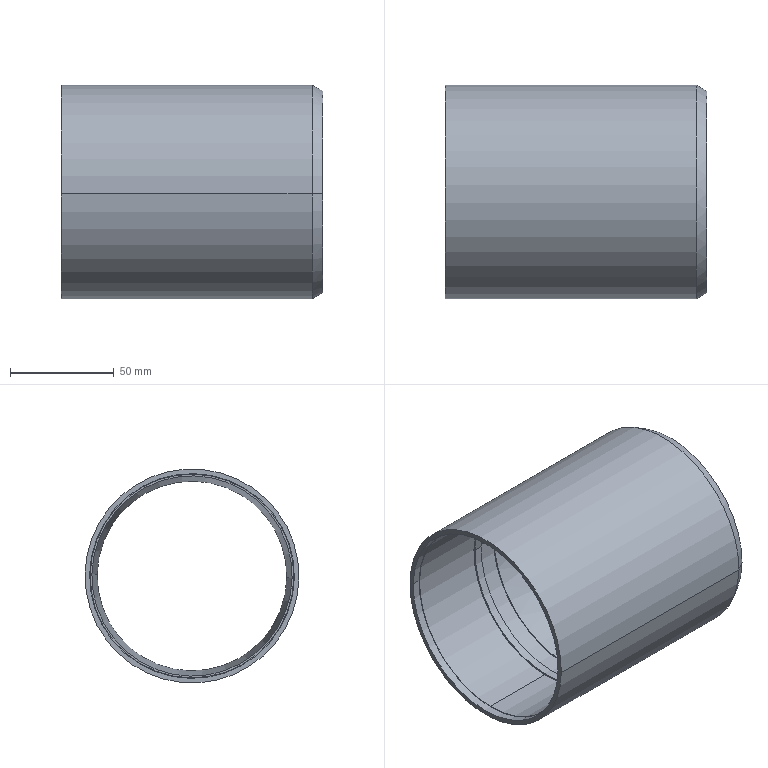Component | SolidWorks | 216InnerTubeAssembly-1_SnapRingSeat-1 | 1 solid | 24 faces | box 126 x 103 x 103 mm | volume 139518 mm3 | cylinder 10 | cone 8 | plane 6 | commonest cylinder face diameters 98.01 x2 98.4 x2 98.539 x2 103 x2 96.4 x2 | material Alloy Steel
build123d program:
from build123d import *

# Parameters (mm, degrees)
SKETCH1_W = 37.278
SKETCH1_H = 1.505


with BuildPart() as part:
    # Model → Revolve1 (revolve)
    with BuildSketch(Plane.XY, mode=Mode.PRIVATE) as revolve1_sk:
        Polygon((-1.168, 45.275), (-0.1676, 46.275), (-0.1676, 48.084), (-5.364, 51.084), (-126.168, 51.084), (-126.168, 48.853), (-122.168, 48.853), (-122.168, 47.784), (-81.168, 47.784), (-81.168, 48.784), (-71.668, 48.784), (-71.668, 48.284), (-8.168, 45.243), align=None)
    revolve(revolve1_sk.sketch.rotate(Axis((-130.696, -0.4163, 0), (1, 0, 0)), 180), axis=Axis((-130.696, -0.4163, 0), (1, 0, 0)))

    # Sketch1 → Cut-Revolve1 (revolve, cut)
    with BuildSketch(Plane.XY, mode=Mode.PRIVATE) as cut_revolve1_sk:
        with Locations((-103.806, 47.836)):
            Rectangle(SKETCH1_W, SKETCH1_H)
    revolve(cut_revolve1_sk.sketch.rotate(Axis((-127.445, -0.4163, 0), (1, 0, 0)), 180), axis=Axis((-127.445, -0.4163, 0), (1, 0, 0)), mode=Mode.SUBTRACT)


solid = part.part

# Placed as in the assembly
solid = solid.moved(Location((2974.445, 0.4163, 0), (0, 0, 0)))
STEP:
#1=CARTESIAN_POINT('',(113.751,0.03464,-1.929));
#2=VERTEX_POINT('',#1);
#3=CARTESIAN_POINT('',(113.751,-0.03464,1.929));
#4=VERTEX_POINT('',#3);
#5=CARTESIAN_POINT('',(113.751,-0.,0.));
#6=DIRECTION('',(-1.,-0.,0.));
#7=DIRECTION('',(0.,-0.01796,0.9998));
#8=AXIS2_PLACEMENT_3D('',#5,#6,#7);
#9=CIRCLE('',#8,1.929);
#10=EDGE_CURVE('',#2,#4,#9,.T.);
#11=ORIENTED_EDGE('',*,*,#10,.F.);
#12=CARTESIAN_POINT('',(112.294,0.03464,-1.929));
#13=VERTEX_POINT('',#12);
#14=CARTESIAN_POINT('',(112.087,0.03464,-1.929));
#15=DIRECTION('',(-1.,-0.,0.));
#16=VECTOR('',#15,39.37);
#17=LINE('',#14,#16);
#18=EDGE_CURVE('',#2,#13,#17,.T.);
#19=ORIENTED_EDGE('',*,*,#18,.T.);
#20=CARTESIAN_POINT('',(112.294,-0.03464,1.929));
#21=VERTEX_POINT('',#20);
#22=CARTESIAN_POINT('',(112.294,-0.,0.));
#23=DIRECTION('',(1.,0.,0.));
#24=DIRECTION('',(0.,-0.9998,-0.01796));
#25=AXIS2_PLACEMENT_3D('',#22,#23,#24);
#26=CIRCLE('',#25,1.929);
#27=EDGE_CURVE('',#21,#13,#26,.T.);
#28=ORIENTED_EDGE('',*,*,#27,.F.);
#29=CARTESIAN_POINT('',(112.087,-0.03464,1.929));
#30=DIRECTION('',(-1.,-0.,0.));
#31=VECTOR('',#30,39.37);
#32=LINE('',#29,#31);
#33=EDGE_CURVE('',#4,#21,#32,.T.);
#34=ORIENTED_EDGE('',*,*,#33,.F.);
#35=EDGE_LOOP('',(#11,#19,#28,#34));
#36=FACE_OUTER_BOUND('',#35,.T.);
#37=CARTESIAN_POINT('',(112.087,-0.,0.));
#38=DIRECTION('',(-1.,-0.,0.));
#39=DIRECTION('',(0.,-0.01796,0.9998));
#40=AXIS2_PLACEMENT_3D('',#37,#38,#39);
#41=CYLINDRICAL_SURFACE('',#40,1.929);
#42=ADVANCED_FACE('',(#36),#41,.F.);
#43=CARTESIAN_POINT('',(116.783,1.797,0.03228));
#44=VERTEX_POINT('',#43);
#45=CARTESIAN_POINT('',(116.783,-1.797,-0.03228));
#46=VERTEX_POINT('',#45);
#47=CARTESIAN_POINT('',(116.783,-0.,0.));
#48=DIRECTION('',(-1.,-0.,-0.));
#49=DIRECTION('',(0.,-0.9998,-0.01796));
#50=AXIS2_PLACEMENT_3D('',#47,#48,#49);
#51=CIRCLE('',#50,1.798);
#52=EDGE_CURVE('',#44,#46,#51,.T.);
#53=ORIENTED_EDGE('',*,*,#52,.T.);
#54=CARTESIAN_POINT('',(117.058,-1.799,-0.0323));
#55=VERTEX_POINT('',#54);
#56=CARTESIAN_POINT('',(116.783,-1.797,-0.03228));
#57=DIRECTION('',(1.,-0.004511,-0.00008102));
#58=VECTOR('',#57,39.37);
#59=LINE('',#56,#58);
#60=EDGE_CURVE('',#46,#55,#59,.T.);
#61=ORIENTED_EDGE('',*,*,#60,.T.);
#62=CARTESIAN_POINT('',(117.058,1.799,0.0323));
#63=VERTEX_POINT('',#62);
#64=CARTESIAN_POINT('',(117.058,-0.,0.));
#65=DIRECTION('',(-1.,-0.,-0.));
#66=DIRECTION('',(0.,-0.9998,-0.01796));
#67=AXIS2_PLACEMENT_3D('',#64,#65,#66);
#68=CIRCLE('',#67,1.799);
#69=EDGE_CURVE('',#63,#55,#68,.T.);
#70=ORIENTED_EDGE('',*,*,#69,.F.);
#71=CARTESIAN_POINT('',(116.783,1.797,0.03228));
#72=DIRECTION('',(1.,0.004511,0.00008102));
#73=VECTOR('',#72,39.37);
#74=LINE('',#71,#73);
#75=EDGE_CURVE('',#44,#63,#74,.T.);
#76=ORIENTED_EDGE('',*,*,#75,.F.);
#77=EDGE_LOOP('',(#53,#61,#70,#76));
#78=FACE_OUTER_BOUND('',#77,.T.);
#79=CARTESIAN_POINT('',(116.783,-0.,0.));
#80=DIRECTION('',(1.,0.,0.));
#81=DIRECTION('',(0.,0.9998,0.01796));
#82=AXIS2_PLACEMENT_3D('',#79,#80,#81);
#83=CONICAL_SURFACE('',#82,1.798,0.004512);
#84=ADVANCED_FACE('',(#78),#83,.F.);
#85=ORIENTED_EDGE('',*,*,#52,.F.);
#86=CARTESIAN_POINT('',(114.283,1.917,0.03443));
#87=VERTEX_POINT('',#86);
#88=CARTESIAN_POINT('',(116.783,1.797,0.03228));
#89=DIRECTION('',(-0.9989,0.04782,0.0008588));
#90=VECTOR('',#89,39.37);
#91=LINE('',#88,#90);
#92=EDGE_CURVE('',#44,#87,#91,.T.);
#93=ORIENTED_EDGE('',*,*,#92,.T.);
#94=CARTESIAN_POINT('',(114.283,-1.917,-0.03443));
#95=VERTEX_POINT('',#94);
#96=CARTESIAN_POINT('',(114.283,-0.,0.));
#97=DIRECTION('',(-1.,-0.,-0.));
#98=DIRECTION('',(0.,-0.9998,-0.01796));
#99=AXIS2_PLACEMENT_3D('',#96,#97,#98);
#100=CIRCLE('',#99,1.917);
#101=EDGE_CURVE('',#87,#95,#100,.T.);
#102=ORIENTED_EDGE('',*,*,#101,.T.);
#103=CARTESIAN_POINT('',(116.783,-1.797,-0.03228));
#104=DIRECTION('',(-0.9989,-0.04782,-0.0008588));
#105=VECTOR('',#104,39.37);
#106=LINE('',#103,#105);
#107=EDGE_CURVE('',#46,#95,#106,.T.);
#108=ORIENTED_EDGE('',*,*,#107,.F.);
#109=EDGE_LOOP('',(#85,#93,#102,#108));
#110=FACE_OUTER_BOUND('',#109,.T.);
#111=CARTESIAN_POINT('',(116.783,-0.,0.));
#112=DIRECTION('',(-1.,-0.,-0.));
#113=DIRECTION('',(0.,-0.9998,-0.01796));
#114=AXIS2_PLACEMENT_3D('',#111,#112,#113);
#115=CONICAL_SURFACE('',#114,1.798,0.04785);
#116=ADVANCED_FACE('',(#110),#115,.F.);
#117=CARTESIAN_POINT('',(114.283,1.937,0.03478));
#118=VERTEX_POINT('',#117);
#119=CARTESIAN_POINT('',(114.283,-1.937,-0.03478));
#120=VERTEX_POINT('',#119);
#121=CARTESIAN_POINT('',(114.283,-0.,0.));
#122=DIRECTION('',(-1.,-0.,-0.));
#123=DIRECTION('',(0.,-0.9998,-0.01796));
#124=AXIS2_PLACEMENT_3D('',#121,#122,#123);
#125=CIRCLE('',#124,1.937);
#126=EDGE_CURVE('',#118,#120,#125,.T.);
#127=ORIENTED_EDGE('',*,*,#126,.F.);
#128=CARTESIAN_POINT('',(113.909,1.937,0.03478));
#129=VERTEX_POINT('',#128);
#130=CARTESIAN_POINT('',(111.959,1.937,0.03478));
#131=DIRECTION('',(-1.,-0.,-0.));
#132=VECTOR('',#131,39.37);
#133=LINE('',#130,#132);
#134=EDGE_CURVE('',#118,#129,#133,.T.);
#135=ORIENTED_EDGE('',*,*,#134,.T.);
#136=CARTESIAN_POINT('',(113.909,-1.937,-0.03478));
#137=VERTEX_POINT('',#136);
#138=CARTESIAN_POINT('',(113.909,-0.,0.));
#139=DIRECTION('',(-1.,-0.,-0.));
#140=DIRECTION('',(0.,-0.9998,-0.01796));
#141=AXIS2_PLACEMENT_3D('',#138,#139,#140);
#142=CIRCLE('',#141,1.937);
#143=EDGE_CURVE('',#129,#137,#142,.T.);
#144=ORIENTED_EDGE('',*,*,#143,.T.);
#145=CARTESIAN_POINT('',(111.959,-1.937,-0.03478));
#146=DIRECTION('',(-1.,-0.,-0.));
#147=VECTOR('',#146,39.37);
#148=LINE('',#145,#147);
#149=EDGE_CURVE('',#120,#137,#148,.T.);
#150=ORIENTED_EDGE('',*,*,#149,.F.);
#151=EDGE_LOOP('',(#127,#135,#144,#150));
#152=FACE_OUTER_BOUND('',#151,.T.);
#153=CARTESIAN_POINT('',(111.959,-0.,0.));
#154=DIRECTION('',(-1.,-0.,-0.));
#155=DIRECTION('',(0.,-0.9998,-0.01796));
#156=AXIS2_PLACEMENT_3D('',#153,#154,#155);
#157=CYLINDRICAL_SURFACE('',#156,1.937);
#158=ADVANCED_FACE('',(#152),#157,.F.);
#159=CARTESIAN_POINT('',(112.294,1.939,0.03483));
#160=VERTEX_POINT('',#159);
#161=CARTESIAN_POINT('',(112.294,-1.939,-0.03483));
#162=VERTEX_POINT('',#161);
#163=CARTESIAN_POINT('',(112.294,-0.,0.));
#164=DIRECTION('',(-1.,-0.,-0.));
#165=DIRECTION('',(0.,-0.9998,-0.01796));
#166=AXIS2_PLACEMENT_3D('',#163,#164,#165);
#167=CIRCLE('',#166,1.94);
#168=EDGE_CURVE('',#160,#162,#167,.T.);
#169=ORIENTED_EDGE('',*,*,#168,.F.);
#170=CARTESIAN_POINT('',(112.137,1.939,0.03483));
#171=VERTEX_POINT('',#170);
#172=CARTESIAN_POINT('',(111.959,1.939,0.03483));
#173=DIRECTION('',(-1.,-0.,-0.));
#174=VECTOR('',#173,39.37);
#175=LINE('',#172,#174);
#176=EDGE_CURVE('',#160,#171,#175,.T.);
#177=ORIENTED_EDGE('',*,*,#176,.T.);
#178=CARTESIAN_POINT('',(112.137,-1.939,-0.03483));
#179=VERTEX_POINT('',#178);
#180=CARTESIAN_POINT('',(112.137,-0.,0.));
#181=DIRECTION('',(-1.,-0.,-0.));
#182=DIRECTION('',(0.,-0.9998,-0.01796));
#183=AXIS2_PLACEMENT_3D('',#180,#181,#182);
#184=CIRCLE('',#183,1.94);
#185=EDGE_CURVE('',#171,#179,#184,.T.);
#186=ORIENTED_EDGE('',*,*,#185,.T.);
#187=CARTESIAN_POINT('',(111.959,-1.939,-0.03483));
#188=DIRECTION('',(-1.,-0.,-0.));
#189=VECTOR('',#188,39.37);
#190=LINE('',#187,#189);
#191=EDGE_CURVE('',#162,#179,#190,.T.);
#192=ORIENTED_EDGE('',*,*,#191,.F.);
#193=EDGE_LOOP('',(#169,#177,#186,#192));
#194=FACE_OUTER_BOUND('',#193,.T.);
#195=CARTESIAN_POINT('',(111.959,-0.,0.));
#196=DIRECTION('',(-1.,-0.,-0.));
#197=DIRECTION('',(0.,-0.9998,-0.01796));
#198=AXIS2_PLACEMENT_3D('',#195,#196,#197);
#199=CYLINDRICAL_SURFACE('',#198,1.94);
#200=ADVANCED_FACE('',(#194),#199,.F.);
#201=CARTESIAN_POINT('',(116.893,-2.027,-0.03641));
#202=VERTEX_POINT('',#201);
#203=CARTESIAN_POINT('',(116.893,2.027,0.03641));
#204=VERTEX_POINT('',#203);
#205=CARTESIAN_POINT('',(116.893,-0.,0.));
#206=DIRECTION('',(-1.,-0.,-0.));
#207=DIRECTION('',(0.,-0.9998,-0.01796));
#208=AXIS2_PLACEMENT_3D('',#205,#206,#207);
#209=CIRCLE('',#208,2.028);
#210=EDGE_CURVE('',#202,#204,#209,.T.);
#211=ORIENTED_EDGE('',*,*,#210,.T.);
#212=CARTESIAN_POINT('',(112.137,2.027,0.03641));
#213=VERTEX_POINT('',#212);
#214=CARTESIAN_POINT('',(111.959,2.027,0.03641));
#215=DIRECTION('',(-1.,-0.,-0.));
#216=VECTOR('',#215,39.37);
#217=LINE('',#214,#216);
#218=EDGE_CURVE('',#204,#213,#217,.T.);
#219=ORIENTED_EDGE('',*,*,#218,.T.);
#220=CARTESIAN_POINT('',(112.137,-2.027,-0.03641));
#221=VERTEX_POINT('',#220);
#222=CARTESIAN_POINT('',(112.137,-0.,0.));
#223=DIRECTION('',(-1.,-0.,-0.));
#224=DIRECTION('',(0.,-0.9998,-0.01796));
#225=AXIS2_PLACEMENT_3D('',#222,#223,#224);
#226=CIRCLE('',#225,2.028);
#227=EDGE_CURVE('',#221,#213,#226,.T.);
#228=ORIENTED_EDGE('',*,*,#227,.F.);
#229=CARTESIAN_POINT('',(111.959,-2.027,-0.03641));
#230=DIRECTION('',(-1.,-0.,-0.));
#231=VECTOR('',#230,39.37);
#232=LINE('',#229,#231);
#233=EDGE_CURVE('',#202,#221,#232,.T.);
#234=ORIENTED_EDGE('',*,*,#233,.F.);
#235=EDGE_LOOP('',(#211,#219,#228,#234));
#236=FACE_OUTER_BOUND('',#235,.T.);
#237=CARTESIAN_POINT('',(111.959,-0.,0.));
#238=DIRECTION('',(-1.,-0.,-0.));
#239=DIRECTION('',(0.,-0.9998,-0.01796));
#240=AXIS2_PLACEMENT_3D('',#237,#238,#239);
#241=CYLINDRICAL_SURFACE('',#240,2.028);
#242=ADVANCED_FACE('',(#236),#241,.T.);
#243=CARTESIAN_POINT('',(117.098,-1.909,-0.03429));
#244=VERTEX_POINT('',#243);
#245=CARTESIAN_POINT('',(117.098,1.909,0.03429));
#246=VERTEX_POINT('',#245);
#247=CARTESIAN_POINT('',(117.098,-0.,0.));
#248=DIRECTION('',(-1.,-0.,-0.));
#249=DIRECTION('',(0.,-0.9998,-0.01796));
#250=AXIS2_PLACEMENT_3D('',#247,#248,#249);
#251=CIRCLE('',#250,1.909);
#252=EDGE_CURVE('',#244,#246,#251,.T.);
#253=ORIENTED_EDGE('',*,*,#252,.T.);
#254=CARTESIAN_POINT('',(117.098,1.909,0.03429));
#255=DIRECTION('',(-0.866,0.4999,0.008978));
#256=VECTOR('',#255,39.37);
#257=LINE('',#254,#256);
#258=EDGE_CURVE('',#246,#204,#257,.T.);
#259=ORIENTED_EDGE('',*,*,#258,.T.);
#260=ORIENTED_EDGE('',*,*,#210,.F.);
#261=CARTESIAN_POINT('',(117.098,-1.909,-0.03429));
#262=DIRECTION('',(-0.866,-0.4999,-0.008978));
#263=VECTOR('',#262,39.37);
#264=LINE('',#261,#263);
#265=EDGE_CURVE('',#244,#202,#264,.T.);
#266=ORIENTED_EDGE('',*,*,#265,.F.);
#267=EDGE_LOOP('',(#253,#259,#260,#266));
#268=FACE_OUTER_BOUND('',#267,.T.);
#269=CARTESIAN_POINT('',(117.098,-0.,0.));
#270=DIRECTION('',(-1.,-0.,-0.));
#271=DIRECTION('',(0.,-0.9998,-0.01796));
#272=AXIS2_PLACEMENT_3D('',#269,#270,#271);
#273=CONICAL_SURFACE('',#272,1.909,0.5236);
#274=ADVANCED_FACE('',(#268),#273,.T.);
#275=ORIENTED_EDGE('',*,*,#69,.T.);
#276=CARTESIAN_POINT('',(117.098,-1.838,-0.03301));
#277=VERTEX_POINT('',#276);
#278=CARTESIAN_POINT('',(117.058,-1.799,-0.0323));
#279=DIRECTION('',(0.7071,-0.707,-0.0127));
#280=VECTOR('',#279,39.37);
#281=LINE('',#278,#280);
#282=EDGE_CURVE('',#55,#277,#281,.T.);
#283=ORIENTED_EDGE('',*,*,#282,.T.);
#284=CARTESIAN_POINT('',(117.098,1.838,0.03301));
#285=VERTEX_POINT('',#284);
#286=CARTESIAN_POINT('',(117.098,-0.,0.));
#287=DIRECTION('',(-1.,-0.,-0.));
#288=DIRECTION('',(0.,-0.9998,-0.01796));
#289=AXIS2_PLACEMENT_3D('',#286,#287,#288);
#290=CIRCLE('',#289,1.838);
#291=EDGE_CURVE('',#285,#277,#290,.T.);
#292=ORIENTED_EDGE('',*,*,#291,.F.);
#293=CARTESIAN_POINT('',(117.058,1.799,0.0323));
#294=DIRECTION('',(0.7071,0.707,0.0127));
#295=VECTOR('',#294,39.37);
#296=LINE('',#293,#295);
#297=EDGE_CURVE('',#63,#285,#296,.T.);
#298=ORIENTED_EDGE('',*,*,#297,.F.);
#299=EDGE_LOOP('',(#275,#283,#292,#298));
#300=FACE_OUTER_BOUND('',#299,.T.);
#301=CARTESIAN_POINT('',(117.058,-0.,0.));
#302=DIRECTION('',(1.,0.,0.));
#303=DIRECTION('',(0.,0.9998,0.01796));
#304=AXIS2_PLACEMENT_3D('',#301,#302,#303);
#305=CONICAL_SURFACE('',#304,1.799,0.7854);
#306=ADVANCED_FACE('',(#300),#305,.F.);
#307=CARTESIAN_POINT('',(113.909,1.897,0.03407));
#308=VERTEX_POINT('',#307);
#309=CARTESIAN_POINT('',(113.909,-1.897,-0.03407));
#310=VERTEX_POINT('',#309);
#311=CARTESIAN_POINT('',(113.909,-0.,0.));
#312=DIRECTION('',(-1.,-0.,-0.));
#313=DIRECTION('',(0.,-0.9998,-0.01796));
#314=AXIS2_PLACEMENT_3D('',#311,#312,#313);
#315=CIRCLE('',#314,1.898);
#316=EDGE_CURVE('',#308,#310,#315,.T.);
#317=ORIENTED_EDGE('',*,*,#316,.F.);
#318=CARTESIAN_POINT('',(113.751,1.897,0.03407));
#319=VERTEX_POINT('',#318);
#320=CARTESIAN_POINT('',(111.959,1.897,0.03407));
#321=DIRECTION('',(-1.,-0.,-0.));
#322=VECTOR('',#321,39.37);
#323=LINE('',#320,#322);
#324=EDGE_CURVE('',#308,#319,#323,.T.);
#325=ORIENTED_EDGE('',*,*,#324,.T.);
#326=CARTESIAN_POINT('',(113.751,-1.897,-0.03407));
#327=VERTEX_POINT('',#326);
#328=CARTESIAN_POINT('',(113.751,-0.,0.));
#329=DIRECTION('',(-1.,-0.,0.));
#330=DIRECTION('',(0.,-0.01796,0.9998));
#331=AXIS2_PLACEMENT_3D('',#328,#329,#330);
#332=CIRCLE('',#331,1.898);
#333=EDGE_CURVE('',#319,#327,#332,.T.);
#334=ORIENTED_EDGE('',*,*,#333,.T.);
#335=CARTESIAN_POINT('',(111.959,-1.897,-0.03407));
#336=DIRECTION('',(-1.,-0.,-0.));
#337=VECTOR('',#336,39.37);
#338=LINE('',#335,#337);
#339=EDGE_CURVE('',#310,#327,#338,.T.);
#340=ORIENTED_EDGE('',*,*,#339,.F.);
#341=EDGE_LOOP('',(#317,#325,#334,#340));
#342=FACE_OUTER_BOUND('',#341,.T.);
#343=CARTESIAN_POINT('',(111.959,-0.,0.));
#344=DIRECTION('',(-1.,-0.,-0.));
#345=DIRECTION('',(0.,-0.9998,-0.01796));
#346=AXIS2_PLACEMENT_3D('',#343,#344,#345);
#347=CYLINDRICAL_SURFACE('',#346,1.898);
#348=ADVANCED_FACE('',(#342),#347,.F.);
#349=ORIENTED_EDGE('',*,*,#324,.F.);
#350=CARTESIAN_POINT('',(113.909,-0.,0.));
#351=DIRECTION('',(-1.,-0.,-0.));
#352=DIRECTION('',(0.,-0.9998,-0.01796));
#353=AXIS2_PLACEMENT_3D('',#350,#351,#352);
#354=CIRCLE('',#353,1.898);
#355=EDGE_CURVE('',#310,#308,#354,.T.);
#356=ORIENTED_EDGE('',*,*,#355,.F.);
#357=ORIENTED_EDGE('',*,*,#339,.T.);
#358=CARTESIAN_POINT('',(113.751,-0.,0.));
#359=DIRECTION('',(-1.,-0.,0.));
#360=DIRECTION('',(0.,-0.01796,0.9998));
#361=AXIS2_PLACEMENT_3D('',#358,#359,#360);
#362=CIRCLE('',#361,1.898);
#363=EDGE_CURVE('',#327,#319,#362,.T.);
#364=ORIENTED_EDGE('',*,*,#363,.T.);
#365=EDGE_LOOP('',(#349,#356,#357,#364));
#366=FACE_OUTER_BOUND('',#365,.T.);
#367=CARTESIAN_POINT('',(111.959,-0.,0.));
#368=DIRECTION('',(-1.,-0.,-0.));
#369=DIRECTION('',(0.,-0.9998,-0.01796));
#370=AXIS2_PLACEMENT_3D('',#367,#368,#369);
#371=CYLINDRICAL_SURFACE('',#370,1.898);
#372=ADVANCED_FACE('',(#366),#371,.F.);
#373=ORIENTED_EDGE('',*,*,#282,.F.);
#374=CARTESIAN_POINT('',(117.058,-0.,0.));
#375=DIRECTION('',(-1.,-0.,-0.));
#376=DIRECTION('',(0.,-0.9998,-0.01796));
#377=AXIS2_PLACEMENT_3D('',#374,#375,#376);
#378=CIRCLE('',#377,1.799);
#379=EDGE_CURVE('',#55,#63,#378,.T.);
#380=ORIENTED_EDGE('',*,*,#379,.T.);
#381=ORIENTED_EDGE('',*,*,#297,.T.);
#382=CARTESIAN_POINT('',(117.098,-0.,0.));
#383=DIRECTION('',(-1.,-0.,-0.));
#384=DIRECTION('',(0.,-0.9998,-0.01796));
#385=AXIS2_PLACEMENT_3D('',#382,#383,#384);
#386=CIRCLE('',#385,1.838);
#387=EDGE_CURVE('',#277,#285,#386,.T.);
#388=ORIENTED_EDGE('',*,*,#387,.F.);
#389=EDGE_LOOP('',(#373,#380,#381,#388));
#390=FACE_OUTER_BOUND('',#389,.T.);
#391=CARTESIAN_POINT('',(117.058,-0.,0.));
#392=DIRECTION('',(1.,0.,0.));
#393=DIRECTION('',(0.,0.9998,0.01796));
#394=AXIS2_PLACEMENT_3D('',#391,#392,#393);
#395=CONICAL_SURFACE('',#394,1.799,0.7854);
#396=ADVANCED_FACE('',(#390),#395,.F.);
#397=ORIENTED_EDGE('',*,*,#252,.F.);
#398=CARTESIAN_POINT('',(117.098,-0.,0.));
#399=DIRECTION('',(-1.,-0.,-0.));
#400=DIRECTION('',(0.,-0.9998,-0.01796));
#401=AXIS2_PLACEMENT_3D('',#398,#399,#400);
#402=CIRCLE('',#401,1.909);
#403=EDGE_CURVE('',#246,#244,#402,.T.);
#404=ORIENTED_EDGE('',*,*,#403,.F.);
#405=EDGE_LOOP('',(#397,#404));
#406=FACE_OUTER_BOUND('',#405,.T.);
#407=ORIENTED_EDGE('',*,*,#291,.T.);
#408=ORIENTED_EDGE('',*,*,#387,.T.);
#409=EDGE_LOOP('',(#407,#408));
#410=FACE_BOUND('',#409,.T.);
#411=CARTESIAN_POINT('',(117.098,0.01639,0.0002943));
#412=DIRECTION('',(-1.,-0.,-0.));
#413=DIRECTION('',(0.,-0.9998,-0.01796));
#414=AXIS2_PLACEMENT_3D('',#411,#412,#413);
#415=PLANE('',#414);
#416=ADVANCED_FACE('',(#406,#410),#415,.F.);
#417=ORIENTED_EDGE('',*,*,#258,.F.);
#418=ORIENTED_EDGE('',*,*,#403,.T.);
#419=ORIENTED_EDGE('',*,*,#265,.T.);
#420=CARTESIAN_POINT('',(116.893,-0.,0.));
#421=DIRECTION('',(-1.,-0.,-0.));
#422=DIRECTION('',(0.,-0.9998,-0.01796));
#423=AXIS2_PLACEMENT_3D('',#420,#421,#422);
#424=CIRCLE('',#423,2.028);
#425=EDGE_CURVE('',#204,#202,#424,.T.);
#426=ORIENTED_EDGE('',*,*,#425,.F.);
#427=EDGE_LOOP('',(#417,#418,#419,#426));
#428=FACE_OUTER_BOUND('',#427,.T.);
#429=CARTESIAN_POINT('',(117.098,-0.,0.));
#430=DIRECTION('',(-1.,-0.,-0.));
#431=DIRECTION('',(0.,-0.9998,-0.01796));
#432=AXIS2_PLACEMENT_3D('',#429,#430,#431);
#433=CONICAL_SURFACE('',#432,1.909,0.5236);
#434=ADVANCED_FACE('',(#428),#433,.T.);
#435=ORIENTED_EDGE('',*,*,#218,.F.);
#436=ORIENTED_EDGE('',*,*,#425,.T.);
#437=ORIENTED_EDGE('',*,*,#233,.T.);
#438=CARTESIAN_POINT('',(112.137,-0.,0.));
#439=DIRECTION('',(-1.,-0.,-0.));
#440=DIRECTION('',(0.,-0.9998,-0.01796));
#441=AXIS2_PLACEMENT_3D('',#438,#439,#440);
#442=CIRCLE('',#441,2.028);
#443=EDGE_CURVE('',#213,#221,#442,.T.);
#444=ORIENTED_EDGE('',*,*,#443,.F.);
#445=EDGE_LOOP('',(#435,#436,#437,#444));
#446=FACE_OUTER_BOUND('',#445,.T.);
#447=CARTESIAN_POINT('',(111.959,-0.,0.));
#448=DIRECTION('',(-1.,-0.,-0.));
#449=DIRECTION('',(0.,-0.9998,-0.01796));
#450=AXIS2_PLACEMENT_3D('',#447,#448,#449);
#451=CYLINDRICAL_SURFACE('',#450,2.028);
#452=ADVANCED_FACE('',(#446),#451,.T.);
#453=CARTESIAN_POINT('',(112.137,-0.,0.));
#454=DIRECTION('',(-1.,-0.,-0.));
#455=DIRECTION('',(0.,-0.9998,-0.01796));
#456=AXIS2_PLACEMENT_3D('',#453,#454,#455);
#457=CIRCLE('',#456,1.94);
#458=EDGE_CURVE('',#179,#171,#457,.T.);
#459=ORIENTED_EDGE('',*,*,#458,.F.);
#460=ORIENTED_EDGE('',*,*,#185,.F.);
#461=EDGE_LOOP('',(#459,#460));
#462=FACE_BOUND('',#461,.T.);
#463=ORIENTED_EDGE('',*,*,#227,.T.);
#464=ORIENTED_EDGE('',*,*,#443,.T.);
#465=EDGE_LOOP('',(#463,#464));
#466=FACE_OUTER_BOUND('',#465,.T.);
#467=CARTESIAN_POINT('',(112.137,0.01639,0.0002943));
#468=DIRECTION('',(1.,0.,0.));
#469=DIRECTION('',(-0.,0.9998,0.01796));
#470=AXIS2_PLACEMENT_3D('',#467,#468,#469);
#471=PLANE('',#470);
#472=ADVANCED_FACE('',(#462,#466),#471,.F.);
#473=ORIENTED_EDGE('',*,*,#176,.F.);
#474=CARTESIAN_POINT('',(112.294,-0.,0.));
#475=DIRECTION('',(-1.,-0.,-0.));
#476=DIRECTION('',(0.,-0.9998,-0.01796));
#477=AXIS2_PLACEMENT_3D('',#474,#475,#476);
#478=CIRCLE('',#477,1.94);
#479=EDGE_CURVE('',#162,#160,#478,.T.);
#480=ORIENTED_EDGE('',*,*,#479,.F.);
#481=ORIENTED_EDGE('',*,*,#191,.T.);
#482=ORIENTED_EDGE('',*,*,#458,.T.);
#483=EDGE_LOOP('',(#473,#480,#481,#482));
#484=FACE_OUTER_BOUND('',#483,.T.);
#485=CARTESIAN_POINT('',(111.959,-0.,0.));
#486=DIRECTION('',(-1.,-0.,-0.));
#487=DIRECTION('',(0.,-0.9998,-0.01796));
#488=AXIS2_PLACEMENT_3D('',#485,#486,#487);
#489=CYLINDRICAL_SURFACE('',#488,1.94);
#490=ADVANCED_FACE('',(#484),#489,.F.);
#491=ORIENTED_EDGE('',*,*,#27,.T.);
#492=CARTESIAN_POINT('',(112.294,-0.,0.));
#493=DIRECTION('',(1.,0.,0.));
#494=DIRECTION('',(0.,-0.9998,-0.01796));
#495=AXIS2_PLACEMENT_3D('',#492,#493,#494);
#496=CIRCLE('',#495,1.929);
#497=EDGE_CURVE('',#13,#21,#496,.T.);
#498=ORIENTED_EDGE('',*,*,#497,.T.);
#499=EDGE_LOOP('',(#491,#498));
#500=FACE_BOUND('',#499,.T.);
#501=ORIENTED_EDGE('',*,*,#479,.T.);
#502=ORIENTED_EDGE('',*,*,#168,.T.);
#503=EDGE_LOOP('',(#501,#502));
#504=FACE_OUTER_BOUND('',#503,.T.);
#505=CARTESIAN_POINT('',(112.294,0.01639,0.0002943));
#506=DIRECTION('',(-1.,-0.,-0.));
#507=DIRECTION('',(0.,-0.9998,-0.01796));
#508=AXIS2_PLACEMENT_3D('',#505,#506,#507);
#509=PLANE('',#508);
#510=ADVANCED_FACE('',(#500,#504),#509,.T.);
#511=ORIENTED_EDGE('',*,*,#355,.T.);
#512=ORIENTED_EDGE('',*,*,#316,.T.);
#513=EDGE_LOOP('',(#511,#512));
#514=FACE_BOUND('',#513,.T.);
#515=CARTESIAN_POINT('',(113.909,-0.,0.));
#516=DIRECTION('',(-1.,-0.,-0.));
#517=DIRECTION('',(0.,-0.9998,-0.01796));
#518=AXIS2_PLACEMENT_3D('',#515,#516,#517);
#519=CIRCLE('',#518,1.937);
#520=EDGE_CURVE('',#137,#129,#519,.T.);
#521=ORIENTED_EDGE('',*,*,#520,.F.);
#522=ORIENTED_EDGE('',*,*,#143,.F.);
#523=EDGE_LOOP('',(#521,#522));
#524=FACE_OUTER_BOUND('',#523,.T.);
#525=CARTESIAN_POINT('',(113.909,0.01639,0.0002943));
#526=DIRECTION('',(1.,0.,0.));
#527=DIRECTION('',(-0.,0.9998,0.01796));
#528=AXIS2_PLACEMENT_3D('',#525,#526,#527);
#529=PLANE('',#528);
#530=ADVANCED_FACE('',(#514,#524),#529,.T.);
#531=ORIENTED_EDGE('',*,*,#134,.F.);
#532=CARTESIAN_POINT('',(114.283,-0.,0.));
#533=DIRECTION('',(-1.,-0.,-0.));
#534=DIRECTION('',(0.,-0.9998,-0.01796));
#535=AXIS2_PLACEMENT_3D('',#532,#533,#534);
#536=CIRCLE('',#535,1.937);
#537=EDGE_CURVE('',#120,#118,#536,.T.);
#538=ORIENTED_EDGE('',*,*,#537,.F.);
#539=ORIENTED_EDGE('',*,*,#149,.T.);
#540=ORIENTED_EDGE('',*,*,#520,.T.);
#541=EDGE_LOOP('',(#531,#538,#539,#540));
#542=FACE_OUTER_BOUND('',#541,.T.);
#543=CARTESIAN_POINT('',(111.959,-0.,0.));
#544=DIRECTION('',(-1.,-0.,-0.));
#545=DIRECTION('',(0.,-0.9998,-0.01796));
#546=AXIS2_PLACEMENT_3D('',#543,#544,#545);
#547=CYLINDRICAL_SURFACE('',#546,1.937);
#548=ADVANCED_FACE('',(#542),#547,.F.);
#549=CARTESIAN_POINT('',(114.283,-0.,0.));
#550=DIRECTION('',(-1.,-0.,-0.));
#551=DIRECTION('',(0.,-0.9998,-0.01796));
#552=AXIS2_PLACEMENT_3D('',#549,#550,#551);
#553=CIRCLE('',#552,1.917);
#554=EDGE_CURVE('',#95,#87,#553,.T.);
#555=ORIENTED_EDGE('',*,*,#554,.F.);
#556=ORIENTED_EDGE('',*,*,#101,.F.);
#557=EDGE_LOOP('',(#555,#556));
#558=FACE_BOUND('',#557,.T.);
#559=ORIENTED_EDGE('',*,*,#537,.T.);
#560=ORIENTED_EDGE('',*,*,#126,.T.);
#561=EDGE_LOOP('',(#559,#560));
#562=FACE_OUTER_BOUND('',#561,.T.);
#563=CARTESIAN_POINT('',(114.283,0.01639,0.0002943));
#564=DIRECTION('',(1.,0.,0.));
#565=DIRECTION('',(-0.,0.9998,0.01796));
#566=AXIS2_PLACEMENT_3D('',#563,#564,#565);
#567=PLANE('',#566);
#568=ADVANCED_FACE('',(#558,#562),#567,.F.);
#569=ORIENTED_EDGE('',*,*,#92,.F.);
#570=CARTESIAN_POINT('',(116.783,-0.,0.));
#571=DIRECTION('',(-1.,-0.,-0.));
#572=DIRECTION('',(0.,-0.9998,-0.01796));
#573=AXIS2_PLACEMENT_3D('',#570,#571,#572);
#574=CIRCLE('',#573,1.798);
#575=EDGE_CURVE('',#46,#44,#574,.T.);
#576=ORIENTED_EDGE('',*,*,#575,.F.);
#577=ORIENTED_EDGE('',*,*,#107,.T.);
#578=ORIENTED_EDGE('',*,*,#554,.T.);
#579=EDGE_LOOP('',(#569,#576,#577,#578));
#580=FACE_OUTER_BOUND('',#579,.T.);
#581=CARTESIAN_POINT('',(116.783,-0.,0.));
#582=DIRECTION('',(-1.,-0.,-0.));
#583=DIRECTION('',(0.,-0.9998,-0.01796));
#584=AXIS2_PLACEMENT_3D('',#581,#582,#583);
#585=CONICAL_SURFACE('',#584,1.798,0.04785);
#586=ADVANCED_FACE('',(#580),#585,.F.);
#587=ORIENTED_EDGE('',*,*,#60,.F.);
#588=ORIENTED_EDGE('',*,*,#575,.T.);
#589=ORIENTED_EDGE('',*,*,#75,.T.);
#590=ORIENTED_EDGE('',*,*,#379,.F.);
#591=EDGE_LOOP('',(#587,#588,#589,#590));
#592=FACE_OUTER_BOUND('',#591,.T.);
#593=CARTESIAN_POINT('',(116.783,-0.,0.));
#594=DIRECTION('',(1.,0.,0.));
#595=DIRECTION('',(0.,0.9998,0.01796));
#596=AXIS2_PLACEMENT_3D('',#593,#594,#595);
#597=CONICAL_SURFACE('',#596,1.798,0.004512);
#598=ADVANCED_FACE('',(#592),#597,.F.);
#599=ORIENTED_EDGE('',*,*,#18,.F.);
#600=CARTESIAN_POINT('',(113.751,-0.,0.));
#601=DIRECTION('',(-1.,-0.,0.));
#602=DIRECTION('',(0.,-0.01796,0.9998));
#603=AXIS2_PLACEMENT_3D('',#600,#601,#602);
#604=CIRCLE('',#603,1.929);
#605=EDGE_CURVE('',#4,#2,#604,.T.);
#606=ORIENTED_EDGE('',*,*,#605,.F.);
#607=ORIENTED_EDGE('',*,*,#33,.T.);
#608=ORIENTED_EDGE('',*,*,#497,.F.);
#609=EDGE_LOOP('',(#599,#606,#607,#608));
#610=FACE_OUTER_BOUND('',#609,.T.);
#611=CARTESIAN_POINT('',(112.087,-0.,0.));
#612=DIRECTION('',(-1.,-0.,0.));
#613=DIRECTION('',(0.,-0.01796,0.9998));
#614=AXIS2_PLACEMENT_3D('',#611,#612,#613);
#615=CYLINDRICAL_SURFACE('',#614,1.929);
#616=ADVANCED_FACE('',(#610),#615,.F.);
#617=ORIENTED_EDGE('',*,*,#363,.F.);
#618=ORIENTED_EDGE('',*,*,#333,.F.);
#619=EDGE_LOOP('',(#617,#618));
#620=FACE_BOUND('',#619,.T.);
#621=ORIENTED_EDGE('',*,*,#605,.T.);
#622=ORIENTED_EDGE('',*,*,#10,.T.);
#623=EDGE_LOOP('',(#621,#622));
#624=FACE_OUTER_BOUND('',#623,.T.);
#625=CARTESIAN_POINT('',(113.751,1.929,0.03464));
#626=DIRECTION('',(-1.,-0.,0.));
#627=DIRECTION('',(0.,-0.01796,0.9998));
#628=AXIS2_PLACEMENT_3D('',#625,#626,#627);
#629=PLANE('',#628);
#630=ADVANCED_FACE('',(#620,#624),#629,.T.);
#631=CLOSED_SHELL('',(#42,#84,#116,#158,#200,#242,#274,#306,#348,#372,#396,#416,#434,#452,#472,#490,#510,#530,#548,#568,#586,#598,#616,#630));
#632=MANIFOLD_SOLID_BREP('',#631);
#633=CARTESIAN_POINT('',(0.,0.,0.));
#634=DIRECTION('',(0.,0.,1.));
#635=DIRECTION('',(1.,0.,0.));
#636=AXIS2_PLACEMENT_3D('',#633,#634,#635);
#637=(LENGTH_UNIT()NAMED_UNIT(*)SI_UNIT($,.METRE.));
#638=LENGTH_MEASURE_WITH_UNIT(LENGTH_MEASURE(0.0254),#637);
#639=DIMENSIONAL_EXPONENTS(1.,0.,0.,0.,0.,0.,0.);
#640=(CONVERSION_BASED_UNIT('',#638)LENGTH_UNIT()NAMED_UNIT(#639));
#641=UNCERTAINTY_MEASURE_WITH_UNIT(LENGTH_MEASURE(0.00001),#640,'','');
#642=(NAMED_UNIT(*)PLANE_ANGLE_UNIT()SI_UNIT($,.RADIAN.));
#643=(NAMED_UNIT(*)SI_UNIT($,.STERADIAN.)SOLID_ANGLE_UNIT());
#644=(GEOMETRIC_REPRESENTATION_CONTEXT(3)GLOBAL_UNCERTAINTY_ASSIGNED_CONTEXT((#641))GLOBAL_UNIT_ASSIGNED_CONTEXT((#640,#642,#643))REPRESENTATION_CONTEXT('',''));
#645=ADVANCED_BREP_SHAPE_REPRESENTATION('',(#632,#636),#644);
#646=COLOUR_RGB('',0.7922,0.8196,0.9333);
#647=FILL_AREA_STYLE_COLOUR('',#646);
#648=FILL_AREA_STYLE('',(#647));
#649=SURFACE_STYLE_FILL_AREA(#648);
#650=SURFACE_SIDE_STYLE('',(#649));
#651=SURFACE_STYLE_USAGE(.BOTH.,#650);
#652=PRESENTATION_STYLE_ASSIGNMENT((#651));
#653=STYLED_ITEM('',(#652),#632);
#654=PRESENTATION_LAYER_ASSIGNMENT('','',(#653));
#655=(LENGTH_UNIT()NAMED_UNIT(*)SI_UNIT($,.METRE.));
#656=LENGTH_MEASURE_WITH_UNIT(LENGTH_MEASURE(0.0254),#655);
#657=DIMENSIONAL_EXPONENTS(1.,0.,0.,0.,0.,0.,0.);
#658=(CONVERSION_BASED_UNIT('',#656)LENGTH_UNIT()NAMED_UNIT(#657));
#659=UNCERTAINTY_MEASURE_WITH_UNIT(LENGTH_MEASURE(0.00001),#658,'','');
#660=(NAMED_UNIT(*)PLANE_ANGLE_UNIT()SI_UNIT($,.RADIAN.));
#661=(NAMED_UNIT(*)SI_UNIT($,.STERADIAN.)SOLID_ANGLE_UNIT());
#662=(GEOMETRIC_REPRESENTATION_CONTEXT(3)GLOBAL_UNCERTAINTY_ASSIGNED_CONTEXT((#659))GLOBAL_UNIT_ASSIGNED_CONTEXT((#658,#660,#661))REPRESENTATION_CONTEXT('',''));
#663=MECHANICAL_DESIGN_GEOMETRIC_PRESENTATION_REPRESENTATION('',(#653),#662);